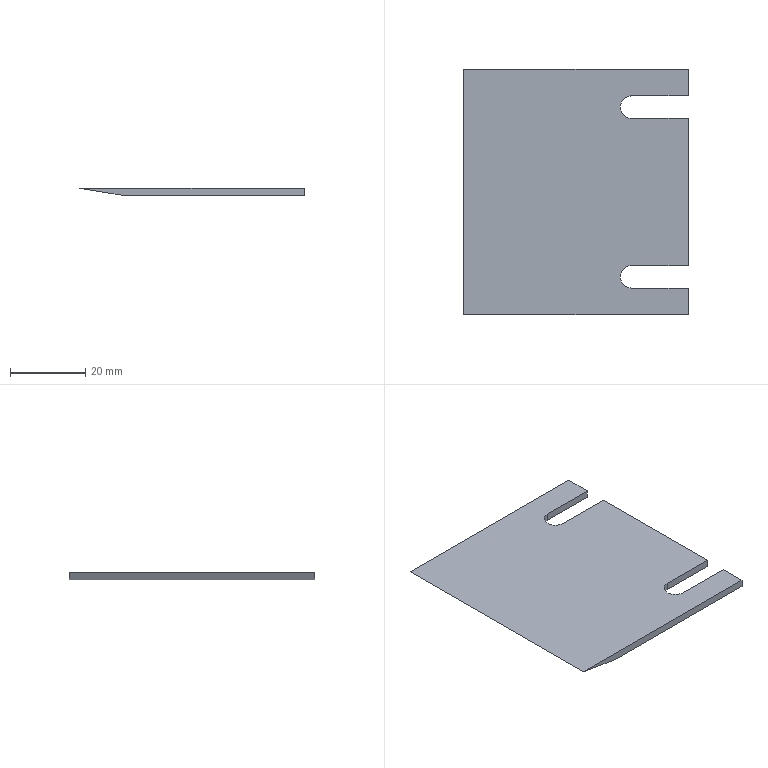Component | SolidWorks | CuttingBladeModification-1 | 1 solid | 14 faces | box 59.5 x 65 x 2 mm | volume 6538 mm3 | plane 12 | cylinder 2 | commonest cylinder face diameters 6 x2
build123d program:
from build123d import *

# Parameters (mm, degrees)
BOSS_EXTRUDE1_DEPTH = 32.5
CUT_EXTRUDE1_DEPTH  = 10


with BuildPart() as part:
    # Sketch1 → Boss-Extrude1 (new, symmetric)
    with BuildSketch(Plane.XY):
        Polygon((-1, 59.5), (1, 59.5), (1, 0), (-1, 12), align=None)
    extrude(amount=BOSS_EXTRUDE1_DEPTH, both=True)

    # Sketch2 → Cut-Extrude1 (cut)
    with BuildSketch(Plane.ZY.offset(1)):
        with BuildLine():
            Line((-25.5, 44.5), (-25.5, 62.94))
            Line((-25.5, 62.94), (-19.5, 62.94))
            Line((-19.5, 62.94), (-19.5, 44.5))
            ThreePointArc((-19.5, 44.5), (-22.5, 41.5), (-25.5, 44.5))
        make_face()
        with BuildLine():
            Line((19.5, 44.5), (19.5, 62.94))
            Line((19.5, 62.94), (25.5, 62.94))
            Line((25.5, 62.94), (25.5, 44.5))
            ThreePointArc((25.5, 44.5), (22.5, 41.5), (19.5, 44.5))
        make_face()
    extrude(amount=-CUT_EXTRUDE1_DEPTH, mode=Mode.SUBTRACT)


solid = part.part

# Placed as in the assembly
solid = solid.moved(Location((-464.272, -281.766, 895.2), (-90, 0, -90)))
STEP:
#1=COLOUR_RGB('',0.7922,0.8196,0.9333);
#2=FILL_AREA_STYLE_COLOUR('',#1);
#3=FILL_AREA_STYLE('',(#2));
#4=SURFACE_STYLE_FILL_AREA(#3);
#5=SURFACE_SIDE_STYLE('',(#4));
#6=SURFACE_STYLE_USAGE(.BOTH.,#5);
#7=PRESENTATION_STYLE_ASSIGNMENT((#6));
#8=CARTESIAN_POINT('',(-15.936,-12.097,35.205));
#9=VERTEX_POINT('',#8);
#10=CARTESIAN_POINT('',(-15.936,-12.373,35.205));
#11=VERTEX_POINT('',#10);
#12=CARTESIAN_POINT('',(-15.936,-9.814,35.205));
#13=DIRECTION('',(0.,-1.,-0.));
#14=VECTOR('',#13,39.37);
#15=LINE('',#12,#14);
#16=EDGE_CURVE('',#9,#11,#15,.T.);
#17=ORIENTED_EDGE('',*,*,#16,.F.);
#18=CARTESIAN_POINT('',(-15.936,-12.097,35.283));
#19=VERTEX_POINT('',#18);
#20=CARTESIAN_POINT('',(-15.936,-12.097,35.205));
#21=DIRECTION('',(-0.,-0.,1.));
#22=VECTOR('',#21,39.37);
#23=LINE('',#20,#22);
#24=EDGE_CURVE('',#9,#19,#23,.T.);
#25=ORIENTED_EDGE('',*,*,#24,.T.);
#26=CARTESIAN_POINT('',(-15.936,-12.373,35.283));
#27=VERTEX_POINT('',#26);
#28=CARTESIAN_POINT('',(-15.936,-9.814,35.283));
#29=DIRECTION('',(0.,-1.,-0.));
#30=VECTOR('',#29,39.37);
#31=LINE('',#28,#30);
#32=EDGE_CURVE('',#19,#27,#31,.T.);
#33=ORIENTED_EDGE('',*,*,#32,.T.);
#34=CARTESIAN_POINT('',(-15.936,-12.373,35.205));
#35=DIRECTION('',(0.,0.,-1.));
#36=VECTOR('',#35,39.37);
#37=LINE('',#34,#36);
#38=EDGE_CURVE('',#27,#11,#37,.T.);
#39=ORIENTED_EDGE('',*,*,#38,.T.);
#40=EDGE_LOOP('',(#17,#25,#33,#39));
#41=FACE_OUTER_BOUND('',#40,.T.);
#42=CARTESIAN_POINT('',(-15.936,-9.814,35.205));
#43=DIRECTION('',(-1.,-0.,-0.));
#44=DIRECTION('',(0.,-1.,-0.));
#45=AXIS2_PLACEMENT_3D('',#42,#43,#44);
#46=PLANE('',#45);
#47=ADVANCED_FACE('',(#41),#46,.F.);
#48=CARTESIAN_POINT('',(-15.936,-9.814,35.283));
#49=VERTEX_POINT('',#48);
#50=CARTESIAN_POINT('',(-15.936,-10.089,35.283));
#51=VERTEX_POINT('',#50);
#52=CARTESIAN_POINT('',(-15.936,-9.814,35.283));
#53=DIRECTION('',(0.,-1.,-0.));
#54=VECTOR('',#53,39.37);
#55=LINE('',#52,#54);
#56=EDGE_CURVE('',#49,#51,#55,.T.);
#57=ORIENTED_EDGE('',*,*,#56,.T.);
#58=CARTESIAN_POINT('',(-15.936,-10.089,35.205));
#59=VERTEX_POINT('',#58);
#60=CARTESIAN_POINT('',(-15.936,-10.089,35.205));
#61=DIRECTION('',(0.,0.,-1.));
#62=VECTOR('',#61,39.37);
#63=LINE('',#60,#62);
#64=EDGE_CURVE('',#51,#59,#63,.T.);
#65=ORIENTED_EDGE('',*,*,#64,.T.);
#66=CARTESIAN_POINT('',(-15.936,-9.814,35.205));
#67=VERTEX_POINT('',#66);
#68=CARTESIAN_POINT('',(-15.936,-9.814,35.205));
#69=DIRECTION('',(0.,-1.,-0.));
#70=VECTOR('',#69,39.37);
#71=LINE('',#68,#70);
#72=EDGE_CURVE('',#67,#59,#71,.T.);
#73=ORIENTED_EDGE('',*,*,#72,.F.);
#74=CARTESIAN_POINT('',(-15.936,-9.814,35.205));
#75=DIRECTION('',(0.,0.,-1.));
#76=VECTOR('',#75,39.37);
#77=LINE('',#74,#76);
#78=EDGE_CURVE('',#49,#67,#77,.T.);
#79=ORIENTED_EDGE('',*,*,#78,.F.);
#80=EDGE_LOOP('',(#57,#65,#73,#79));
#81=FACE_OUTER_BOUND('',#80,.T.);
#82=CARTESIAN_POINT('',(-15.936,-9.814,35.205));
#83=DIRECTION('',(-1.,-0.,-0.));
#84=DIRECTION('',(0.,-1.,-0.));
#85=AXIS2_PLACEMENT_3D('',#82,#83,#84);
#86=PLANE('',#85);
#87=ADVANCED_FACE('',(#81),#86,.F.);
#88=CARTESIAN_POINT('',(-16.526,-12.097,35.205));
#89=VERTEX_POINT('',#88);
#90=CARTESIAN_POINT('',(-16.526,-11.861,35.205));
#91=VERTEX_POINT('',#90);
#92=CARTESIAN_POINT('',(-16.526,-11.979,35.205));
#93=DIRECTION('',(0.,0.,-1.));
#94=DIRECTION('',(0.,1.,0.));
#95=AXIS2_PLACEMENT_3D('',#92,#93,#94);
#96=CIRCLE('',#95,0.1181);
#97=EDGE_CURVE('',#89,#91,#96,.T.);
#98=ORIENTED_EDGE('',*,*,#97,.F.);
#99=CARTESIAN_POINT('',(-16.526,-12.097,35.205));
#100=DIRECTION('',(-1.,-0.,-0.));
#101=VECTOR('',#100,39.37);
#102=LINE('',#99,#101);
#103=EDGE_CURVE('',#9,#89,#102,.T.);
#104=ORIENTED_EDGE('',*,*,#103,.F.);
#105=ORIENTED_EDGE('',*,*,#16,.T.);
#106=CARTESIAN_POINT('',(-17.806,-12.373,35.205));
#107=VERTEX_POINT('',#106);
#108=CARTESIAN_POINT('',(-15.936,-12.373,35.205));
#109=DIRECTION('',(-1.,-0.,-0.));
#110=VECTOR('',#109,39.37);
#111=LINE('',#108,#110);
#112=EDGE_CURVE('',#11,#107,#111,.T.);
#113=ORIENTED_EDGE('',*,*,#112,.T.);
#114=CARTESIAN_POINT('',(-17.806,-9.814,35.205));
#115=VERTEX_POINT('',#114);
#116=CARTESIAN_POINT('',(-17.806,-9.814,35.205));
#117=DIRECTION('',(0.,-1.,-0.));
#118=VECTOR('',#117,39.37);
#119=LINE('',#116,#118);
#120=EDGE_CURVE('',#115,#107,#119,.T.);
#121=ORIENTED_EDGE('',*,*,#120,.F.);
#122=CARTESIAN_POINT('',(-15.936,-9.814,35.205));
#123=DIRECTION('',(-1.,-0.,-0.));
#124=VECTOR('',#123,39.37);
#125=LINE('',#122,#124);
#126=EDGE_CURVE('',#67,#115,#125,.T.);
#127=ORIENTED_EDGE('',*,*,#126,.F.);
#128=ORIENTED_EDGE('',*,*,#72,.T.);
#129=CARTESIAN_POINT('',(-16.526,-10.089,35.205));
#130=VERTEX_POINT('',#129);
#131=CARTESIAN_POINT('',(-16.526,-10.089,35.205));
#132=DIRECTION('',(1.,0.,0.));
#133=VECTOR('',#132,39.37);
#134=LINE('',#131,#133);
#135=EDGE_CURVE('',#130,#59,#134,.T.);
#136=ORIENTED_EDGE('',*,*,#135,.F.);
#137=CARTESIAN_POINT('',(-16.526,-10.325,35.205));
#138=VERTEX_POINT('',#137);
#139=CARTESIAN_POINT('',(-16.526,-10.207,35.205));
#140=DIRECTION('',(0.,0.,-1.));
#141=DIRECTION('',(0.,1.,0.));
#142=AXIS2_PLACEMENT_3D('',#139,#140,#141);
#143=CIRCLE('',#142,0.1181);
#144=EDGE_CURVE('',#138,#130,#143,.T.);
#145=ORIENTED_EDGE('',*,*,#144,.F.);
#146=CARTESIAN_POINT('',(-15.936,-10.325,35.205));
#147=VERTEX_POINT('',#146);
#148=CARTESIAN_POINT('',(-16.526,-10.325,35.205));
#149=DIRECTION('',(-1.,-0.,-0.));
#150=VECTOR('',#149,39.37);
#151=LINE('',#148,#150);
#152=EDGE_CURVE('',#147,#138,#151,.T.);
#153=ORIENTED_EDGE('',*,*,#152,.F.);
#154=CARTESIAN_POINT('',(-15.936,-11.861,35.205));
#155=VERTEX_POINT('',#154);
#156=CARTESIAN_POINT('',(-15.936,-9.814,35.205));
#157=DIRECTION('',(0.,-1.,-0.));
#158=VECTOR('',#157,39.37);
#159=LINE('',#156,#158);
#160=EDGE_CURVE('',#147,#155,#159,.T.);
#161=ORIENTED_EDGE('',*,*,#160,.T.);
#162=CARTESIAN_POINT('',(-16.526,-11.861,35.205));
#163=DIRECTION('',(1.,0.,0.));
#164=VECTOR('',#163,39.37);
#165=LINE('',#162,#164);
#166=EDGE_CURVE('',#91,#155,#165,.T.);
#167=ORIENTED_EDGE('',*,*,#166,.F.);
#168=EDGE_LOOP('',(#98,#104,#105,#113,#121,#127,#128,#136,#145,#153,#161,#167));
#169=FACE_OUTER_BOUND('',#168,.T.);
#170=CARTESIAN_POINT('',(-15.936,-9.814,35.205));
#171=DIRECTION('',(-0.,-0.,1.));
#172=DIRECTION('',(1.,0.,0.));
#173=AXIS2_PLACEMENT_3D('',#170,#171,#172);
#174=PLANE('',#173);
#175=ADVANCED_FACE('',(#169),#174,.F.);
#176=CARTESIAN_POINT('',(-18.278,-12.373,35.283));
#177=VERTEX_POINT('',#176);
#178=CARTESIAN_POINT('',(-17.806,-12.373,35.205));
#179=DIRECTION('',(-0.9864,-0.,0.1644));
#180=VECTOR('',#179,39.37);
#181=LINE('',#178,#180);
#182=EDGE_CURVE('',#107,#177,#181,.T.);
#183=ORIENTED_EDGE('',*,*,#182,.T.);
#184=CARTESIAN_POINT('',(-18.278,-9.814,35.283));
#185=VERTEX_POINT('',#184);
#186=CARTESIAN_POINT('',(-18.278,-9.814,35.283));
#187=DIRECTION('',(0.,-1.,-0.));
#188=VECTOR('',#187,39.37);
#189=LINE('',#186,#188);
#190=EDGE_CURVE('',#185,#177,#189,.T.);
#191=ORIENTED_EDGE('',*,*,#190,.F.);
#192=CARTESIAN_POINT('',(-17.806,-9.814,35.205));
#193=DIRECTION('',(-0.9864,-0.,0.1644));
#194=VECTOR('',#193,39.37);
#195=LINE('',#192,#194);
#196=EDGE_CURVE('',#115,#185,#195,.T.);
#197=ORIENTED_EDGE('',*,*,#196,.F.);
#198=ORIENTED_EDGE('',*,*,#120,.T.);
#199=EDGE_LOOP('',(#183,#191,#197,#198));
#200=FACE_OUTER_BOUND('',#199,.T.);
#201=CARTESIAN_POINT('',(-17.806,-9.814,35.205));
#202=DIRECTION('',(0.1644,-0.,0.9864));
#203=DIRECTION('',(0.9864,0.,-0.1644));
#204=AXIS2_PLACEMENT_3D('',#201,#202,#203);
#205=PLANE('',#204);
#206=ADVANCED_FACE('',(#200),#205,.F.);
#207=ORIENTED_EDGE('',*,*,#32,.F.);
#208=CARTESIAN_POINT('',(-16.526,-12.097,35.283));
#209=VERTEX_POINT('',#208);
#210=CARTESIAN_POINT('',(-15.936,-12.097,35.283));
#211=DIRECTION('',(-1.,-0.,-0.));
#212=VECTOR('',#211,39.37);
#213=LINE('',#210,#212);
#214=EDGE_CURVE('',#19,#209,#213,.T.);
#215=ORIENTED_EDGE('',*,*,#214,.T.);
#216=CARTESIAN_POINT('',(-16.526,-11.861,35.283));
#217=VERTEX_POINT('',#216);
#218=CARTESIAN_POINT('',(-16.526,-11.979,35.283));
#219=DIRECTION('',(0.,0.,-1.));
#220=DIRECTION('',(-1.,0.,0.));
#221=AXIS2_PLACEMENT_3D('',#218,#219,#220);
#222=CIRCLE('',#221,0.1181);
#223=EDGE_CURVE('',#209,#217,#222,.T.);
#224=ORIENTED_EDGE('',*,*,#223,.T.);
#225=CARTESIAN_POINT('',(-15.936,-11.861,35.283));
#226=VERTEX_POINT('',#225);
#227=CARTESIAN_POINT('',(-15.936,-11.861,35.283));
#228=DIRECTION('',(1.,0.,0.));
#229=VECTOR('',#228,39.37);
#230=LINE('',#227,#229);
#231=EDGE_CURVE('',#217,#226,#230,.T.);
#232=ORIENTED_EDGE('',*,*,#231,.T.);
#233=CARTESIAN_POINT('',(-15.936,-10.325,35.283));
#234=VERTEX_POINT('',#233);
#235=CARTESIAN_POINT('',(-15.936,-9.814,35.283));
#236=DIRECTION('',(0.,-1.,-0.));
#237=VECTOR('',#236,39.37);
#238=LINE('',#235,#237);
#239=EDGE_CURVE('',#234,#226,#238,.T.);
#240=ORIENTED_EDGE('',*,*,#239,.F.);
#241=CARTESIAN_POINT('',(-16.526,-10.325,35.283));
#242=VERTEX_POINT('',#241);
#243=CARTESIAN_POINT('',(-15.936,-10.325,35.283));
#244=DIRECTION('',(-1.,-0.,-0.));
#245=VECTOR('',#244,39.37);
#246=LINE('',#243,#245);
#247=EDGE_CURVE('',#234,#242,#246,.T.);
#248=ORIENTED_EDGE('',*,*,#247,.T.);
#249=CARTESIAN_POINT('',(-16.526,-10.089,35.283));
#250=VERTEX_POINT('',#249);
#251=CARTESIAN_POINT('',(-16.526,-10.207,35.283));
#252=DIRECTION('',(0.,0.,-1.));
#253=DIRECTION('',(-1.,0.,0.));
#254=AXIS2_PLACEMENT_3D('',#251,#252,#253);
#255=CIRCLE('',#254,0.1181);
#256=EDGE_CURVE('',#242,#250,#255,.T.);
#257=ORIENTED_EDGE('',*,*,#256,.T.);
#258=CARTESIAN_POINT('',(-15.936,-10.089,35.283));
#259=DIRECTION('',(1.,0.,0.));
#260=VECTOR('',#259,39.37);
#261=LINE('',#258,#260);
#262=EDGE_CURVE('',#250,#51,#261,.T.);
#263=ORIENTED_EDGE('',*,*,#262,.T.);
#264=ORIENTED_EDGE('',*,*,#56,.F.);
#265=CARTESIAN_POINT('',(-15.936,-9.814,35.283));
#266=DIRECTION('',(1.,0.,0.));
#267=VECTOR('',#266,39.37);
#268=LINE('',#265,#267);
#269=EDGE_CURVE('',#185,#49,#268,.T.);
#270=ORIENTED_EDGE('',*,*,#269,.F.);
#271=ORIENTED_EDGE('',*,*,#190,.T.);
#272=CARTESIAN_POINT('',(-15.936,-12.373,35.283));
#273=DIRECTION('',(1.,0.,0.));
#274=VECTOR('',#273,39.37);
#275=LINE('',#272,#274);
#276=EDGE_CURVE('',#177,#27,#275,.T.);
#277=ORIENTED_EDGE('',*,*,#276,.T.);
#278=EDGE_LOOP('',(#207,#215,#224,#232,#240,#248,#257,#263,#264,#270,#271,#277));
#279=FACE_OUTER_BOUND('',#278,.T.);
#280=CARTESIAN_POINT('',(-15.936,-9.814,35.283));
#281=DIRECTION('',(0.,0.,-1.));
#282=DIRECTION('',(-1.,-0.,-0.));
#283=AXIS2_PLACEMENT_3D('',#280,#281,#282);
#284=PLANE('',#283);
#285=ADVANCED_FACE('',(#279),#284,.F.);
#286=ORIENTED_EDGE('',*,*,#239,.T.);
#287=CARTESIAN_POINT('',(-15.936,-11.861,35.205));
#288=DIRECTION('',(0.,0.,-1.));
#289=VECTOR('',#288,39.37);
#290=LINE('',#287,#289);
#291=EDGE_CURVE('',#226,#155,#290,.T.);
#292=ORIENTED_EDGE('',*,*,#291,.T.);
#293=ORIENTED_EDGE('',*,*,#160,.F.);
#294=CARTESIAN_POINT('',(-15.936,-10.325,35.205));
#295=DIRECTION('',(-0.,-0.,1.));
#296=VECTOR('',#295,39.37);
#297=LINE('',#294,#296);
#298=EDGE_CURVE('',#147,#234,#297,.T.);
#299=ORIENTED_EDGE('',*,*,#298,.T.);
#300=EDGE_LOOP('',(#286,#292,#293,#299));
#301=FACE_OUTER_BOUND('',#300,.T.);
#302=CARTESIAN_POINT('',(-15.936,-9.814,35.205));
#303=DIRECTION('',(-1.,-0.,-0.));
#304=DIRECTION('',(0.,-1.,-0.));
#305=AXIS2_PLACEMENT_3D('',#302,#303,#304);
#306=PLANE('',#305);
#307=ADVANCED_FACE('',(#301),#306,.F.);
#308=ORIENTED_EDGE('',*,*,#126,.T.);
#309=ORIENTED_EDGE('',*,*,#196,.T.);
#310=ORIENTED_EDGE('',*,*,#269,.T.);
#311=ORIENTED_EDGE('',*,*,#78,.T.);
#312=EDGE_LOOP('',(#308,#309,#310,#311));
#313=FACE_OUTER_BOUND('',#312,.T.);
#314=CARTESIAN_POINT('',(-18.278,-9.814,35.244));
#315=DIRECTION('',(-0.,1.,0.));
#316=DIRECTION('',(-0.,-0.,1.));
#317=AXIS2_PLACEMENT_3D('',#314,#315,#316);
#318=PLANE('',#317);
#319=ADVANCED_FACE('',(#313),#318,.T.);
#320=ORIENTED_EDGE('',*,*,#112,.F.);
#321=ORIENTED_EDGE('',*,*,#38,.F.);
#322=ORIENTED_EDGE('',*,*,#276,.F.);
#323=ORIENTED_EDGE('',*,*,#182,.F.);
#324=EDGE_LOOP('',(#320,#321,#322,#323));
#325=FACE_OUTER_BOUND('',#324,.T.);
#326=CARTESIAN_POINT('',(-18.278,-12.373,35.244));
#327=DIRECTION('',(-0.,1.,0.));
#328=DIRECTION('',(-0.,-0.,1.));
#329=AXIS2_PLACEMENT_3D('',#326,#327,#328);
#330=PLANE('',#329);
#331=ADVANCED_FACE('',(#325),#330,.F.);
#332=CARTESIAN_POINT('',(-16.526,-10.325,35.598));
#333=DIRECTION('',(0.,0.,-1.));
#334=VECTOR('',#333,39.37);
#335=LINE('',#332,#334);
#336=EDGE_CURVE('',#242,#138,#335,.T.);
#337=ORIENTED_EDGE('',*,*,#336,.T.);
#338=ORIENTED_EDGE('',*,*,#144,.T.);
#339=CARTESIAN_POINT('',(-16.526,-10.089,35.598));
#340=DIRECTION('',(0.,0.,-1.));
#341=VECTOR('',#340,39.37);
#342=LINE('',#339,#341);
#343=EDGE_CURVE('',#250,#130,#342,.T.);
#344=ORIENTED_EDGE('',*,*,#343,.F.);
#345=ORIENTED_EDGE('',*,*,#256,.F.);
#346=EDGE_LOOP('',(#337,#338,#344,#345));
#347=FACE_OUTER_BOUND('',#346,.T.);
#348=CARTESIAN_POINT('',(-16.526,-10.207,35.598));
#349=DIRECTION('',(0.,0.,-1.));
#350=DIRECTION('',(0.,1.,0.));
#351=AXIS2_PLACEMENT_3D('',#348,#349,#350);
#352=CYLINDRICAL_SURFACE('',#351,0.1181);
#353=ADVANCED_FACE('',(#347),#352,.F.);
#354=ORIENTED_EDGE('',*,*,#343,.T.);
#355=ORIENTED_EDGE('',*,*,#135,.T.);
#356=ORIENTED_EDGE('',*,*,#64,.F.);
#357=ORIENTED_EDGE('',*,*,#262,.F.);
#358=EDGE_LOOP('',(#354,#355,#356,#357));
#359=FACE_OUTER_BOUND('',#358,.T.);
#360=CARTESIAN_POINT('',(-16.526,-10.089,35.598));
#361=DIRECTION('',(-0.,1.,0.));
#362=DIRECTION('',(-0.,-0.,1.));
#363=AXIS2_PLACEMENT_3D('',#360,#361,#362);
#364=PLANE('',#363);
#365=ADVANCED_FACE('',(#359),#364,.F.);
#366=ORIENTED_EDGE('',*,*,#298,.F.);
#367=ORIENTED_EDGE('',*,*,#152,.T.);
#368=ORIENTED_EDGE('',*,*,#336,.F.);
#369=ORIENTED_EDGE('',*,*,#247,.F.);
#370=EDGE_LOOP('',(#366,#367,#368,#369));
#371=FACE_OUTER_BOUND('',#370,.T.);
#372=CARTESIAN_POINT('',(-16.526,-10.325,35.598));
#373=DIRECTION('',(0.,-1.,-0.));
#374=DIRECTION('',(0.,0.,-1.));
#375=AXIS2_PLACEMENT_3D('',#372,#373,#374);
#376=PLANE('',#375);
#377=ADVANCED_FACE('',(#371),#376,.F.);
#378=CARTESIAN_POINT('',(-16.526,-12.097,35.598));
#379=DIRECTION('',(0.,0.,-1.));
#380=VECTOR('',#379,39.37);
#381=LINE('',#378,#380);
#382=EDGE_CURVE('',#209,#89,#381,.T.);
#383=ORIENTED_EDGE('',*,*,#382,.T.);
#384=ORIENTED_EDGE('',*,*,#97,.T.);
#385=CARTESIAN_POINT('',(-16.526,-11.861,35.598));
#386=DIRECTION('',(0.,0.,-1.));
#387=VECTOR('',#386,39.37);
#388=LINE('',#385,#387);
#389=EDGE_CURVE('',#217,#91,#388,.T.);
#390=ORIENTED_EDGE('',*,*,#389,.F.);
#391=ORIENTED_EDGE('',*,*,#223,.F.);
#392=EDGE_LOOP('',(#383,#384,#390,#391));
#393=FACE_OUTER_BOUND('',#392,.T.);
#394=CARTESIAN_POINT('',(-16.526,-11.979,35.598));
#395=DIRECTION('',(0.,0.,-1.));
#396=DIRECTION('',(0.,1.,0.));
#397=AXIS2_PLACEMENT_3D('',#394,#395,#396);
#398=CYLINDRICAL_SURFACE('',#397,0.1181);
#399=ADVANCED_FACE('',(#393),#398,.F.);
#400=ORIENTED_EDGE('',*,*,#24,.F.);
#401=ORIENTED_EDGE('',*,*,#103,.T.);
#402=ORIENTED_EDGE('',*,*,#382,.F.);
#403=ORIENTED_EDGE('',*,*,#214,.F.);
#404=EDGE_LOOP('',(#400,#401,#402,#403));
#405=FACE_OUTER_BOUND('',#404,.T.);
#406=CARTESIAN_POINT('',(-16.526,-12.097,35.598));
#407=DIRECTION('',(0.,-1.,-0.));
#408=DIRECTION('',(0.,0.,-1.));
#409=AXIS2_PLACEMENT_3D('',#406,#407,#408);
#410=PLANE('',#409);
#411=ADVANCED_FACE('',(#405),#410,.F.);
#412=ORIENTED_EDGE('',*,*,#389,.T.);
#413=ORIENTED_EDGE('',*,*,#166,.T.);
#414=ORIENTED_EDGE('',*,*,#291,.F.);
#415=ORIENTED_EDGE('',*,*,#231,.F.);
#416=EDGE_LOOP('',(#412,#413,#414,#415));
#417=FACE_OUTER_BOUND('',#416,.T.);
#418=CARTESIAN_POINT('',(-16.526,-11.861,35.598));
#419=DIRECTION('',(-0.,1.,0.));
#420=DIRECTION('',(-0.,-0.,1.));
#421=AXIS2_PLACEMENT_3D('',#418,#419,#420);
#422=PLANE('',#421);
#423=ADVANCED_FACE('',(#417),#422,.F.);
#424=CLOSED_SHELL('',(#47,#87,#175,#206,#285,#307,#319,#331,#353,#365,#377,#399,#411,#423));
#425=MANIFOLD_SOLID_BREP('',#424);
#426=STYLED_ITEM('',(#7),#425);
#427=PRESENTATION_LAYER_ASSIGNMENT('','',(#426));
#428=CARTESIAN_POINT('',(0.,0.,0.));
#429=DIRECTION('',(0.,0.,1.));
#430=DIRECTION('',(1.,0.,0.));
#431=AXIS2_PLACEMENT_3D('',#428,#429,#430);
#432=(LENGTH_UNIT()NAMED_UNIT(*)SI_UNIT($,.METRE.));
#433=LENGTH_MEASURE_WITH_UNIT(LENGTH_MEASURE(0.0254),#432);
#434=DIMENSIONAL_EXPONENTS(1.,0.,0.,0.,0.,0.,0.);
#435=(CONVERSION_BASED_UNIT('',#433)LENGTH_UNIT()NAMED_UNIT(#434));
#436=UNCERTAINTY_MEASURE_WITH_UNIT(LENGTH_MEASURE(0.00001),#435,'','');
#437=(NAMED_UNIT(*)PLANE_ANGLE_UNIT()SI_UNIT($,.RADIAN.));
#438=(NAMED_UNIT(*)SI_UNIT($,.STERADIAN.)SOLID_ANGLE_UNIT());
#439=(GEOMETRIC_REPRESENTATION_CONTEXT(3)GLOBAL_UNCERTAINTY_ASSIGNED_CONTEXT((#436))GLOBAL_UNIT_ASSIGNED_CONTEXT((#435,#437,#438))REPRESENTATION_CONTEXT('',''));
#440=ADVANCED_BREP_SHAPE_REPRESENTATION('',(#425,#431),#439);
#441=(LENGTH_UNIT()NAMED_UNIT(*)SI_UNIT($,.METRE.));
#442=LENGTH_MEASURE_WITH_UNIT(LENGTH_MEASURE(0.0254),#441);
#443=DIMENSIONAL_EXPONENTS(1.,0.,0.,0.,0.,0.,0.);
#444=(CONVERSION_BASED_UNIT('',#442)LENGTH_UNIT()NAMED_UNIT(#443));
#445=UNCERTAINTY_MEASURE_WITH_UNIT(LENGTH_MEASURE(0.00001),#444,'','');
#446=(NAMED_UNIT(*)PLANE_ANGLE_UNIT()SI_UNIT($,.RADIAN.));
#447=(NAMED_UNIT(*)SI_UNIT($,.STERADIAN.)SOLID_ANGLE_UNIT());
#448=(GEOMETRIC_REPRESENTATION_CONTEXT(3)GLOBAL_UNCERTAINTY_ASSIGNED_CONTEXT((#445))GLOBAL_UNIT_ASSIGNED_CONTEXT((#444,#446,#447))REPRESENTATION_CONTEXT('',''));
#449=MECHANICAL_DESIGN_GEOMETRIC_PRESENTATION_REPRESENTATION('',(#426),#448);